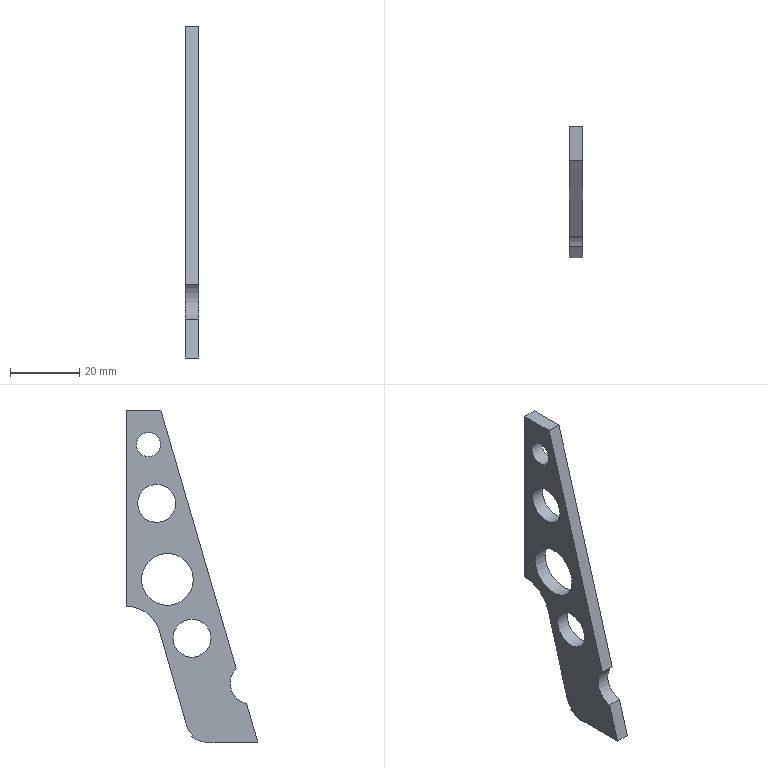Component | NX | 02B__27_2 | 1 solid | 17 faces | volume 5462 mm3 | plane 9 | cylinder 8 | commonest cylinder face diameters 12 x2 11 x2 7 x1 15 x1 10 x1 20 x1